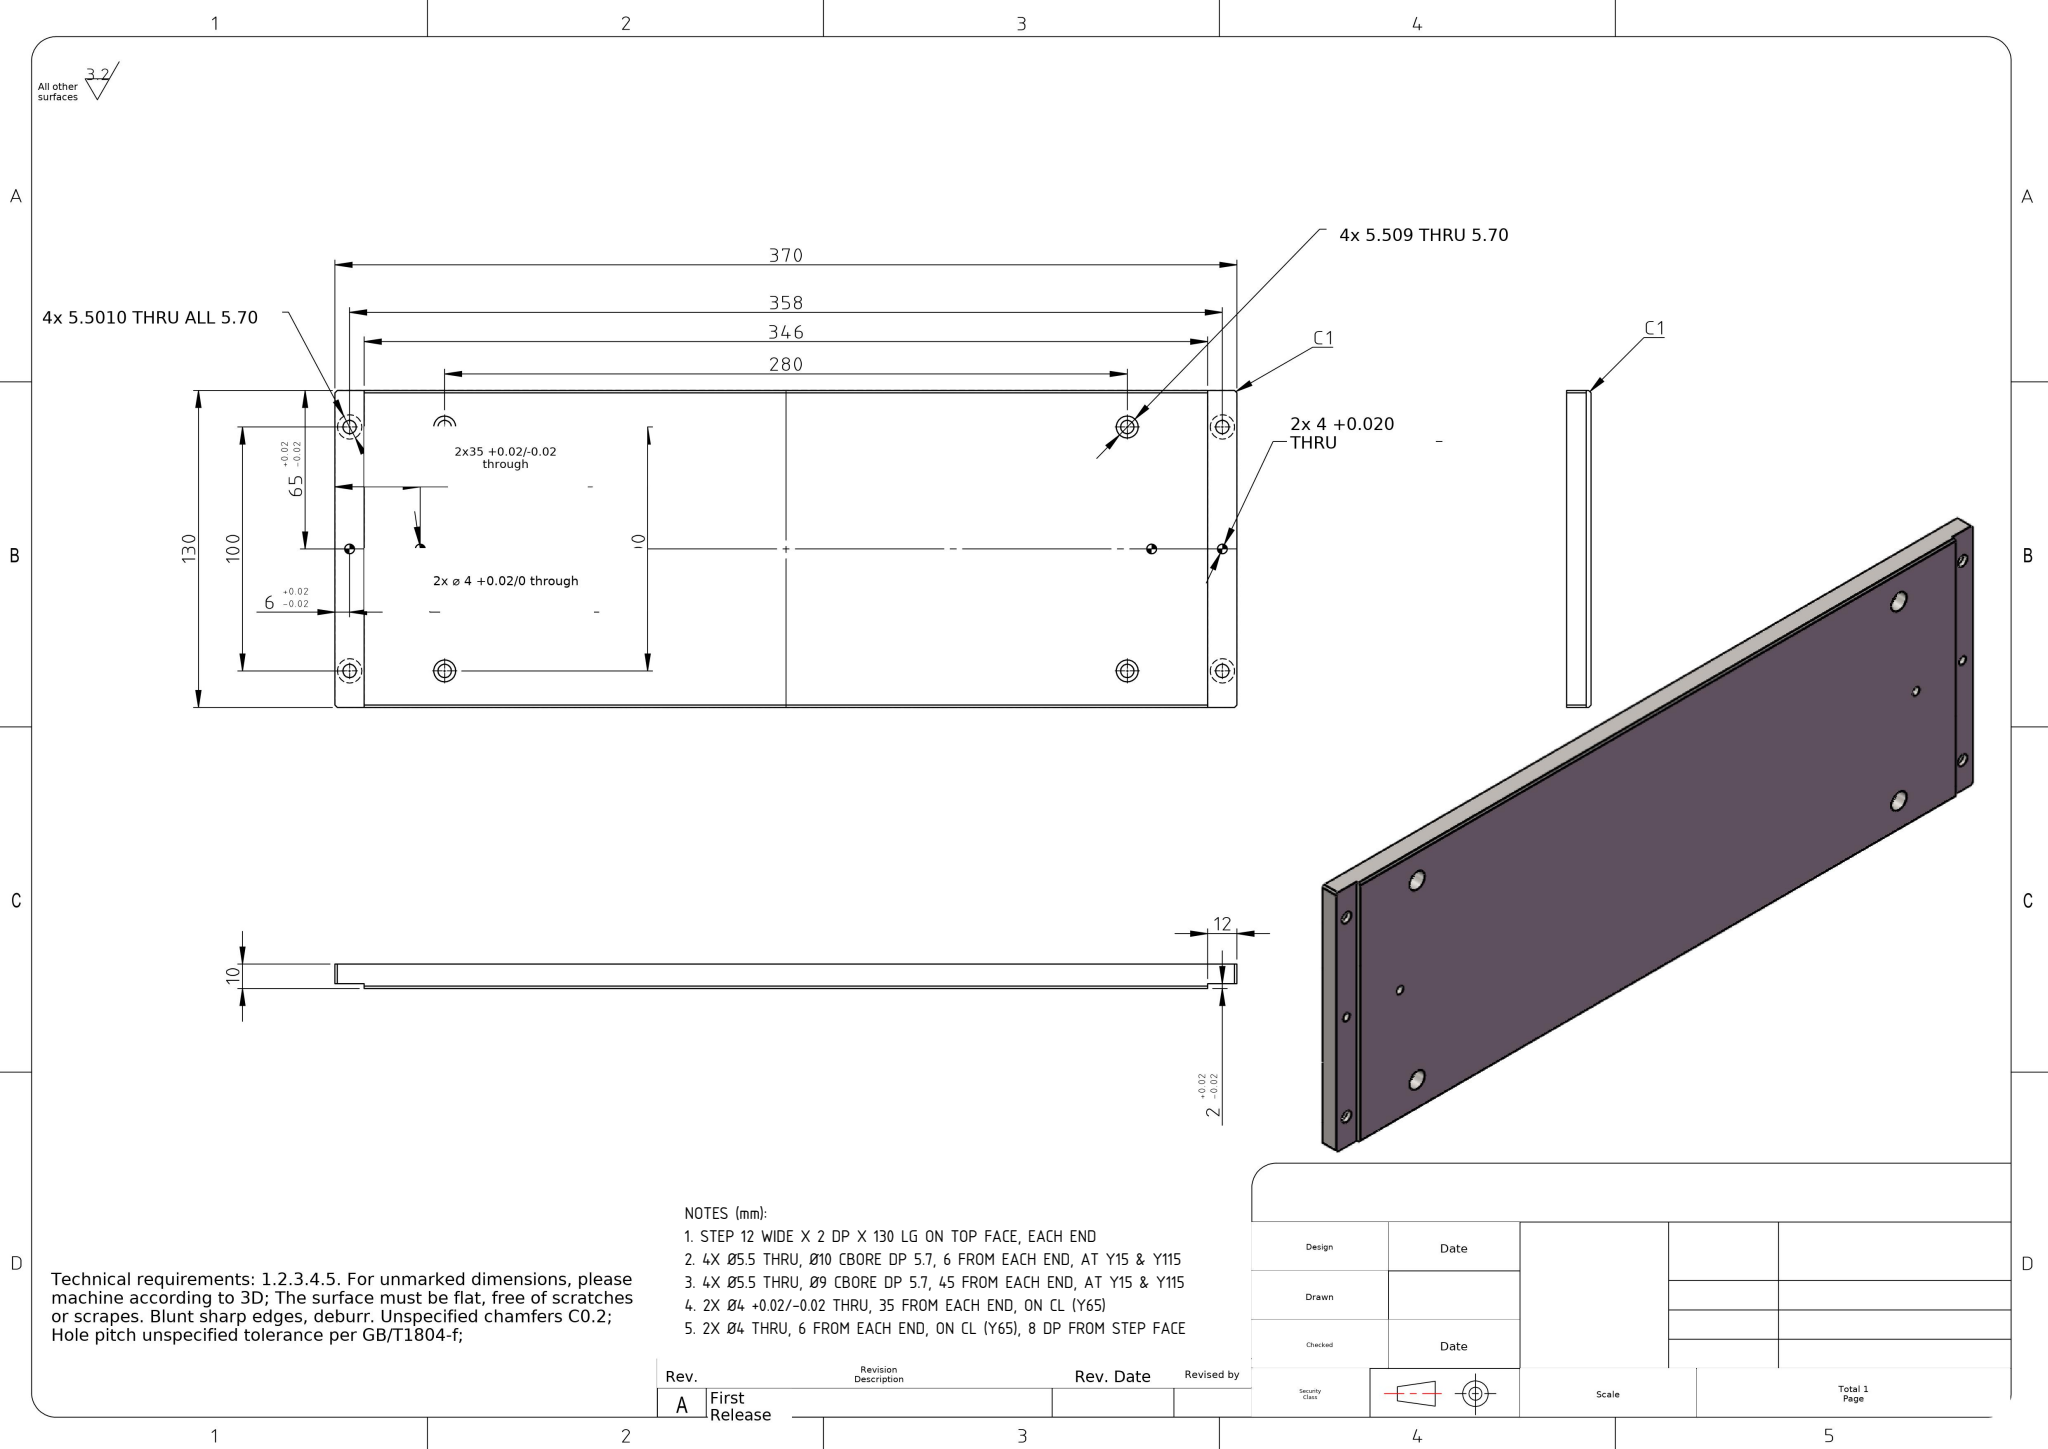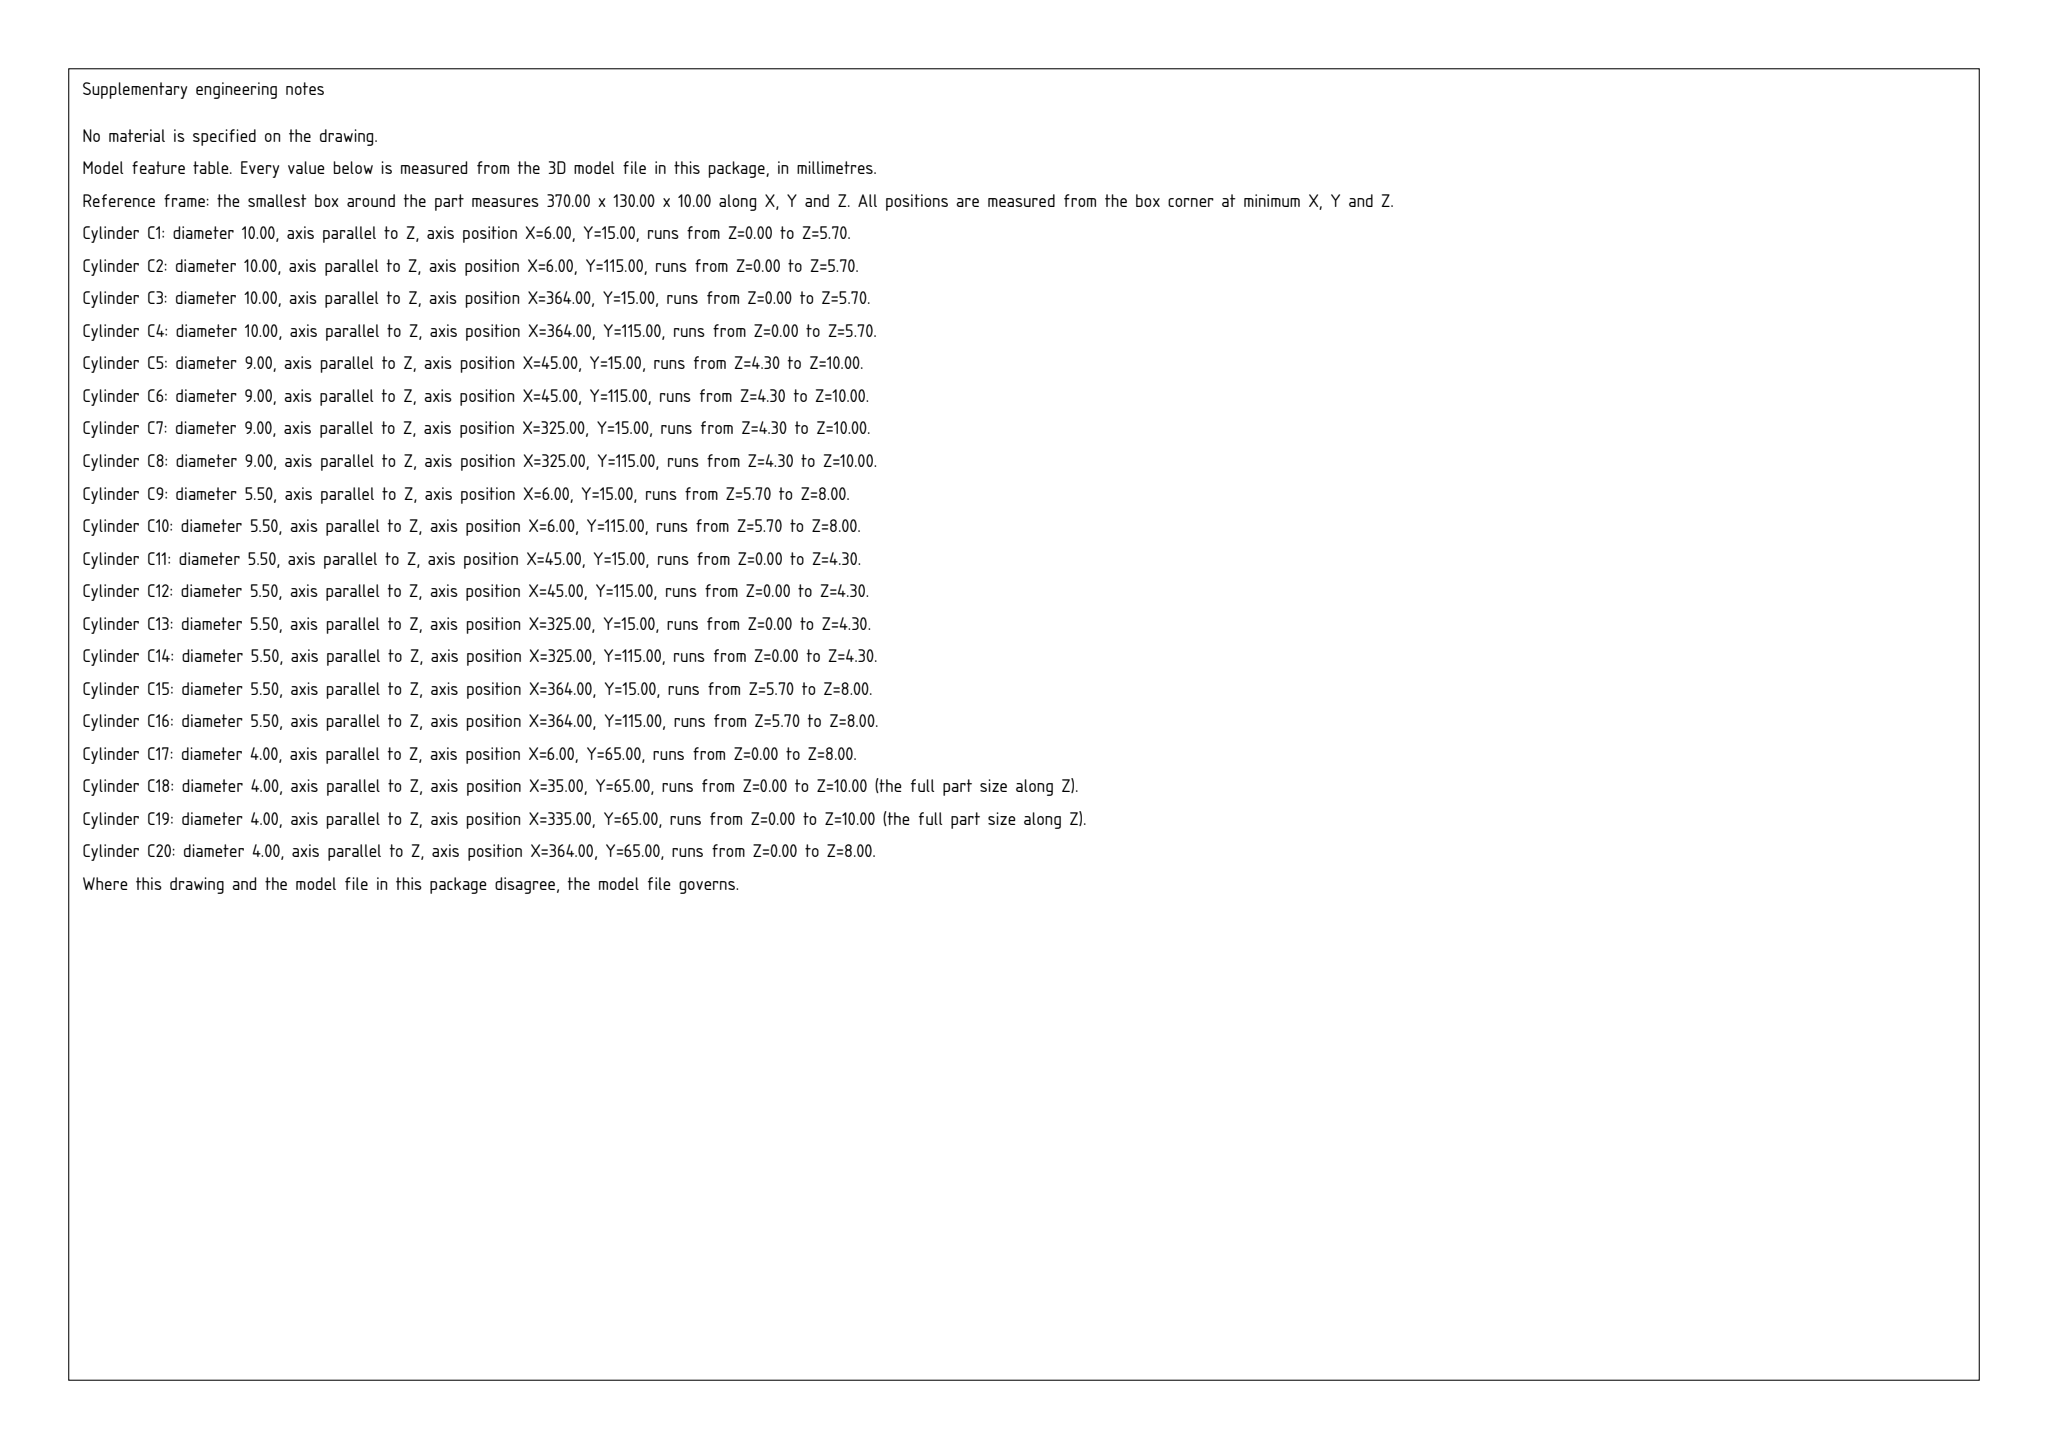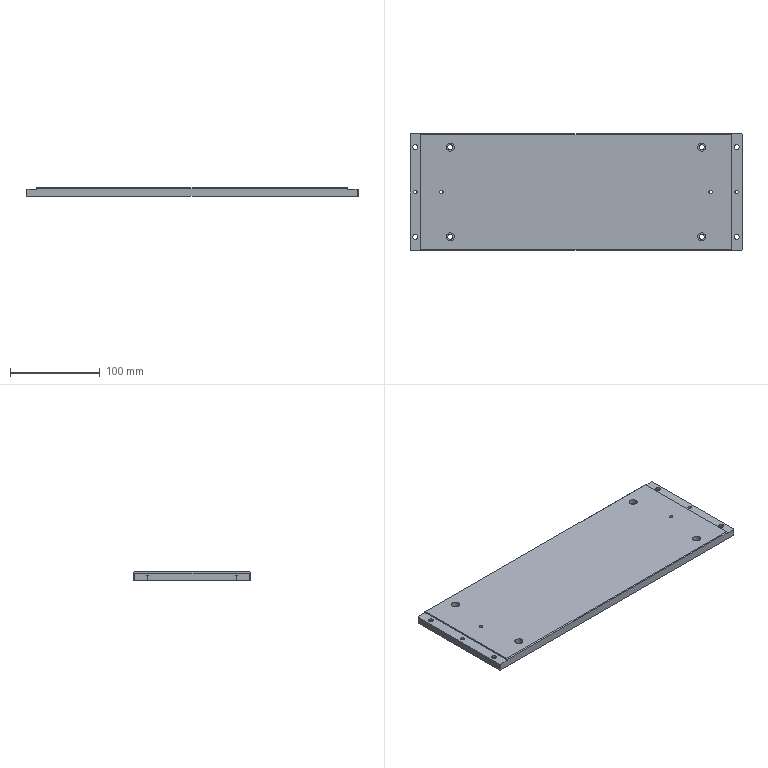Part | SolidWorks | mm | 1 solid | 64 faces | box 370 x 130 x 10 mm | volume 470077 mm3 | cylinder 40 | plane 24 | commonest cylinder face diameters 5.5 x16 4 x8 9 x8 10 x8
Drawing notes:
STEP 12 WIDE X 2 DP X 130 LG ON TOP FACE, EACH END | from the solid: x-planes 0/12 & 358/370; z-plane 8.0 (2 faces) vs top 10.0; bbox Y=130
4X Ø5.5 THRU, Ø10 CBORE DP 5.7, 6 FROM EACH END, AT Y15 & Y115 | from the solid: Ø5.5 L2.3 at [6,15],[6,115],[364,15],[364,115] coaxial w/ Ø10 L5.7; 2.3+5.7=8 step thk
4X Ø5.5 THRU, Ø9 CBORE DP 5.7, 45 FROM EACH END, AT Y15 & Y115 | from the solid: Ø5.5 L4.3 at [45,15],[45,115],[325,15],[325,115] coaxial w/ Ø9 L5.7; 4.3+5.7=10 plate thk
2X Ø4 +0.02/-0.02 THRU, 35 FROM EACH END, ON CL (Y65) | from the solid: Ø4 z-axis cyls at [35,65] and [335,65], L10 thru plate
2X Ø4 THRU, 6 FROM EACH END, ON CL (Y65), 8 DP FROM STEP FACE | from the solid: Ø4 z-axis cyls at [6,65] and [364,65], L8 = plate 10 less 2 step
build123d program:
from build123d import *

# Parameters (mm, degrees)
SKETCH1_W                                         = 370
SKETCH1_H                                         = 130
BOSS_EXTRUDE1_DEPTH                               = 5
SKETCH2_W                                         = 48.158
SKETCH2_H                                         = 130
CUT_EXTRUDE1_DEPTH                                = 2
HOLE_SIZE_ACCORDING_TO_HEXAGON_SOCKET_D           = 5.5
HOLE_SIZE_ACCORDING_TO_HEXAGON_SOCKET_CBORE_D     = 10
HOLE_SIZE_ACCORDING_TO_HEXAGON_SOCKET_CBORE_DEPTH = 5.7
CHAMFER1_SIZE                                     = 1
HOLE_SIZE_ACCORDING_TO_SLOTTED_PAN_HE_D           = 5.5
HOLE_SIZE_ACCORDING_TO_SLOTTED_PAN_HE_CBORE_D     = 9
HOLE_SIZE_ACCORDING_TO_SLOTTED_PAN_HE_CBORE_DEPTH = 5.7
SIZE_MM_DOWEL_PIN_HOLE_1_D                        = 4
SIZE_MM_DOWEL_PIN_HOLE_2_D                        = 4


with BuildPart() as part:
    # Sketch1 → Boss-Extrude1 (new, symmetric)
    with BuildSketch(Plane.XY):
        Rectangle(SKETCH1_W, SKETCH1_H)
    extrude(amount=BOSS_EXTRUDE1_DEPTH, both=True)

    # Sketch2 → Cut-Extrude1 (cut)
    with BuildSketch(Plane.XY.offset(5)):
        with Locations((-197.079, 0)):
            Rectangle(SKETCH2_W, SKETCH2_H)
    cut_extrude1 = extrude(amount=-CUT_EXTRUDE1_DEPTH, mode=Mode.SUBTRACT)

    # Mirror1: Cut-Extrude1 across plane
    add(cut_extrude1.mirror(Plane(origin=(0, 0, 0), x_dir=(0, 0, 1), z_dir=(1, 0, 0))), mode=Mode.SUBTRACT)

    # Hole Size _ according to_ Hexagon Socket (through all)
    with Locations(Plane(origin=(0, 0, -5), x_dir=(-1, 0, 0), z_dir=(0, 0, -1))):
        with Locations((179, -50), (179, 50), (-179, -50), (-179, 50)):
            CounterBoreHole(HOLE_SIZE_ACCORDING_TO_HEXAGON_SOCKET_D / 2, HOLE_SIZE_ACCORDING_TO_HEXAGON_SOCKET_CBORE_D / 2, HOLE_SIZE_ACCORDING_TO_HEXAGON_SOCKET_CBORE_DEPTH)

    # Chamfer1
    chamfer1_edges = [part.edges().sort_by_distance(p)[0] for p in [
        (0, -65, 5),
        (-185, -65, -1),
        (-185, 65, -1),
        (0, 65, 5),
        (185, -65, -1),
        (185, 65, -1),
    ]]
    chamfer(chamfer1_edges, length=CHAMFER1_SIZE)

    # Hole Size _ according to_ Slotted Pan He (through all)
    with Locations(Plane.XY.offset(5)):
        with Locations((-140, 50), (-140, -50), (140, -50), (140, 50)):
            CounterBoreHole(HOLE_SIZE_ACCORDING_TO_SLOTTED_PAN_HE_D / 2, HOLE_SIZE_ACCORDING_TO_SLOTTED_PAN_HE_CBORE_D / 2, HOLE_SIZE_ACCORDING_TO_SLOTTED_PAN_HE_CBORE_DEPTH)

    # Size mm Dowel Pin Hole 1 (through all)
    with Locations(Plane.XY.offset(5)):
        with Locations((-150, 0), (150, 0)):
            Hole(SIZE_MM_DOWEL_PIN_HOLE_1_D / 2)

    # Size mm Dowel Pin Hole 2 (through all)
    with Locations(Plane(origin=(0, 0, -5), x_dir=(-1, 0, 0), z_dir=(0, 0, -1))):
        with Locations((179, 0), (-179, 0)):
            Hole(SIZE_MM_DOWEL_PIN_HOLE_2_D / 2)


solid = part.part